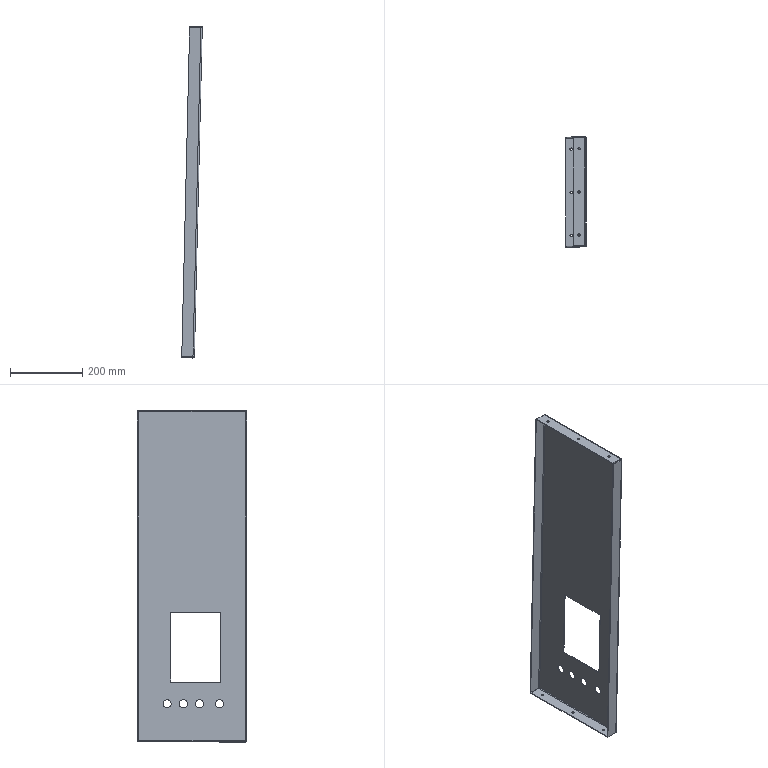Component | SolidWorks | 2403MA0512-1 | 1 solid | 62 faces | volume 654441 mm3 | cylinder 28 | plane 26 | spline 8 | commonest cylinder face diameters 6.6 x12 22.5 x8 8 x4 4 x4 | material SUS304